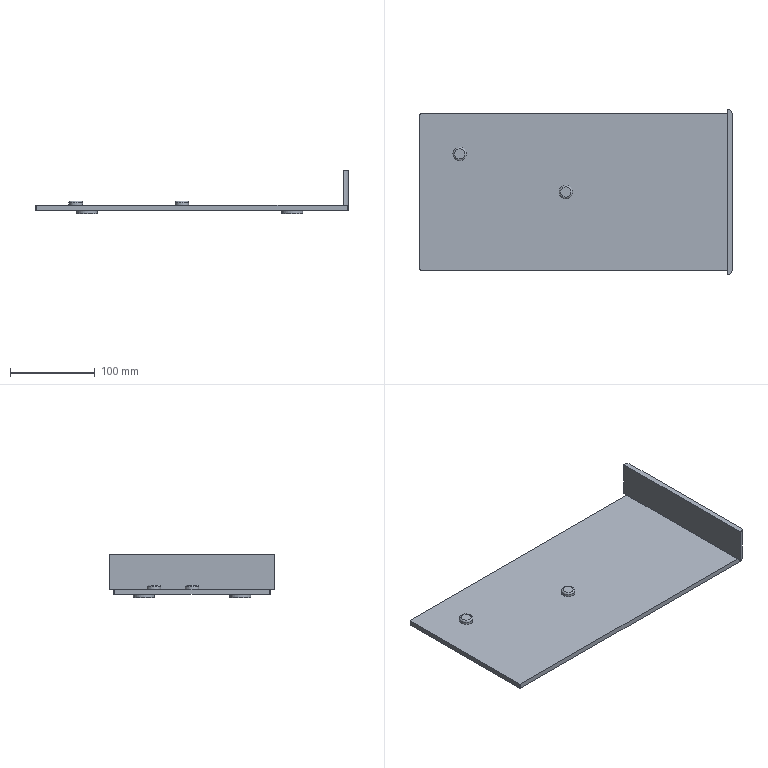Component | NX | L_BASE | 1 solid | 30 faces | volume 463864 mm3 | plane 16 | cylinder 12 | torus 2 | commonest cylinder face diameters 25 x4 2 x4 16 x2 12 x2